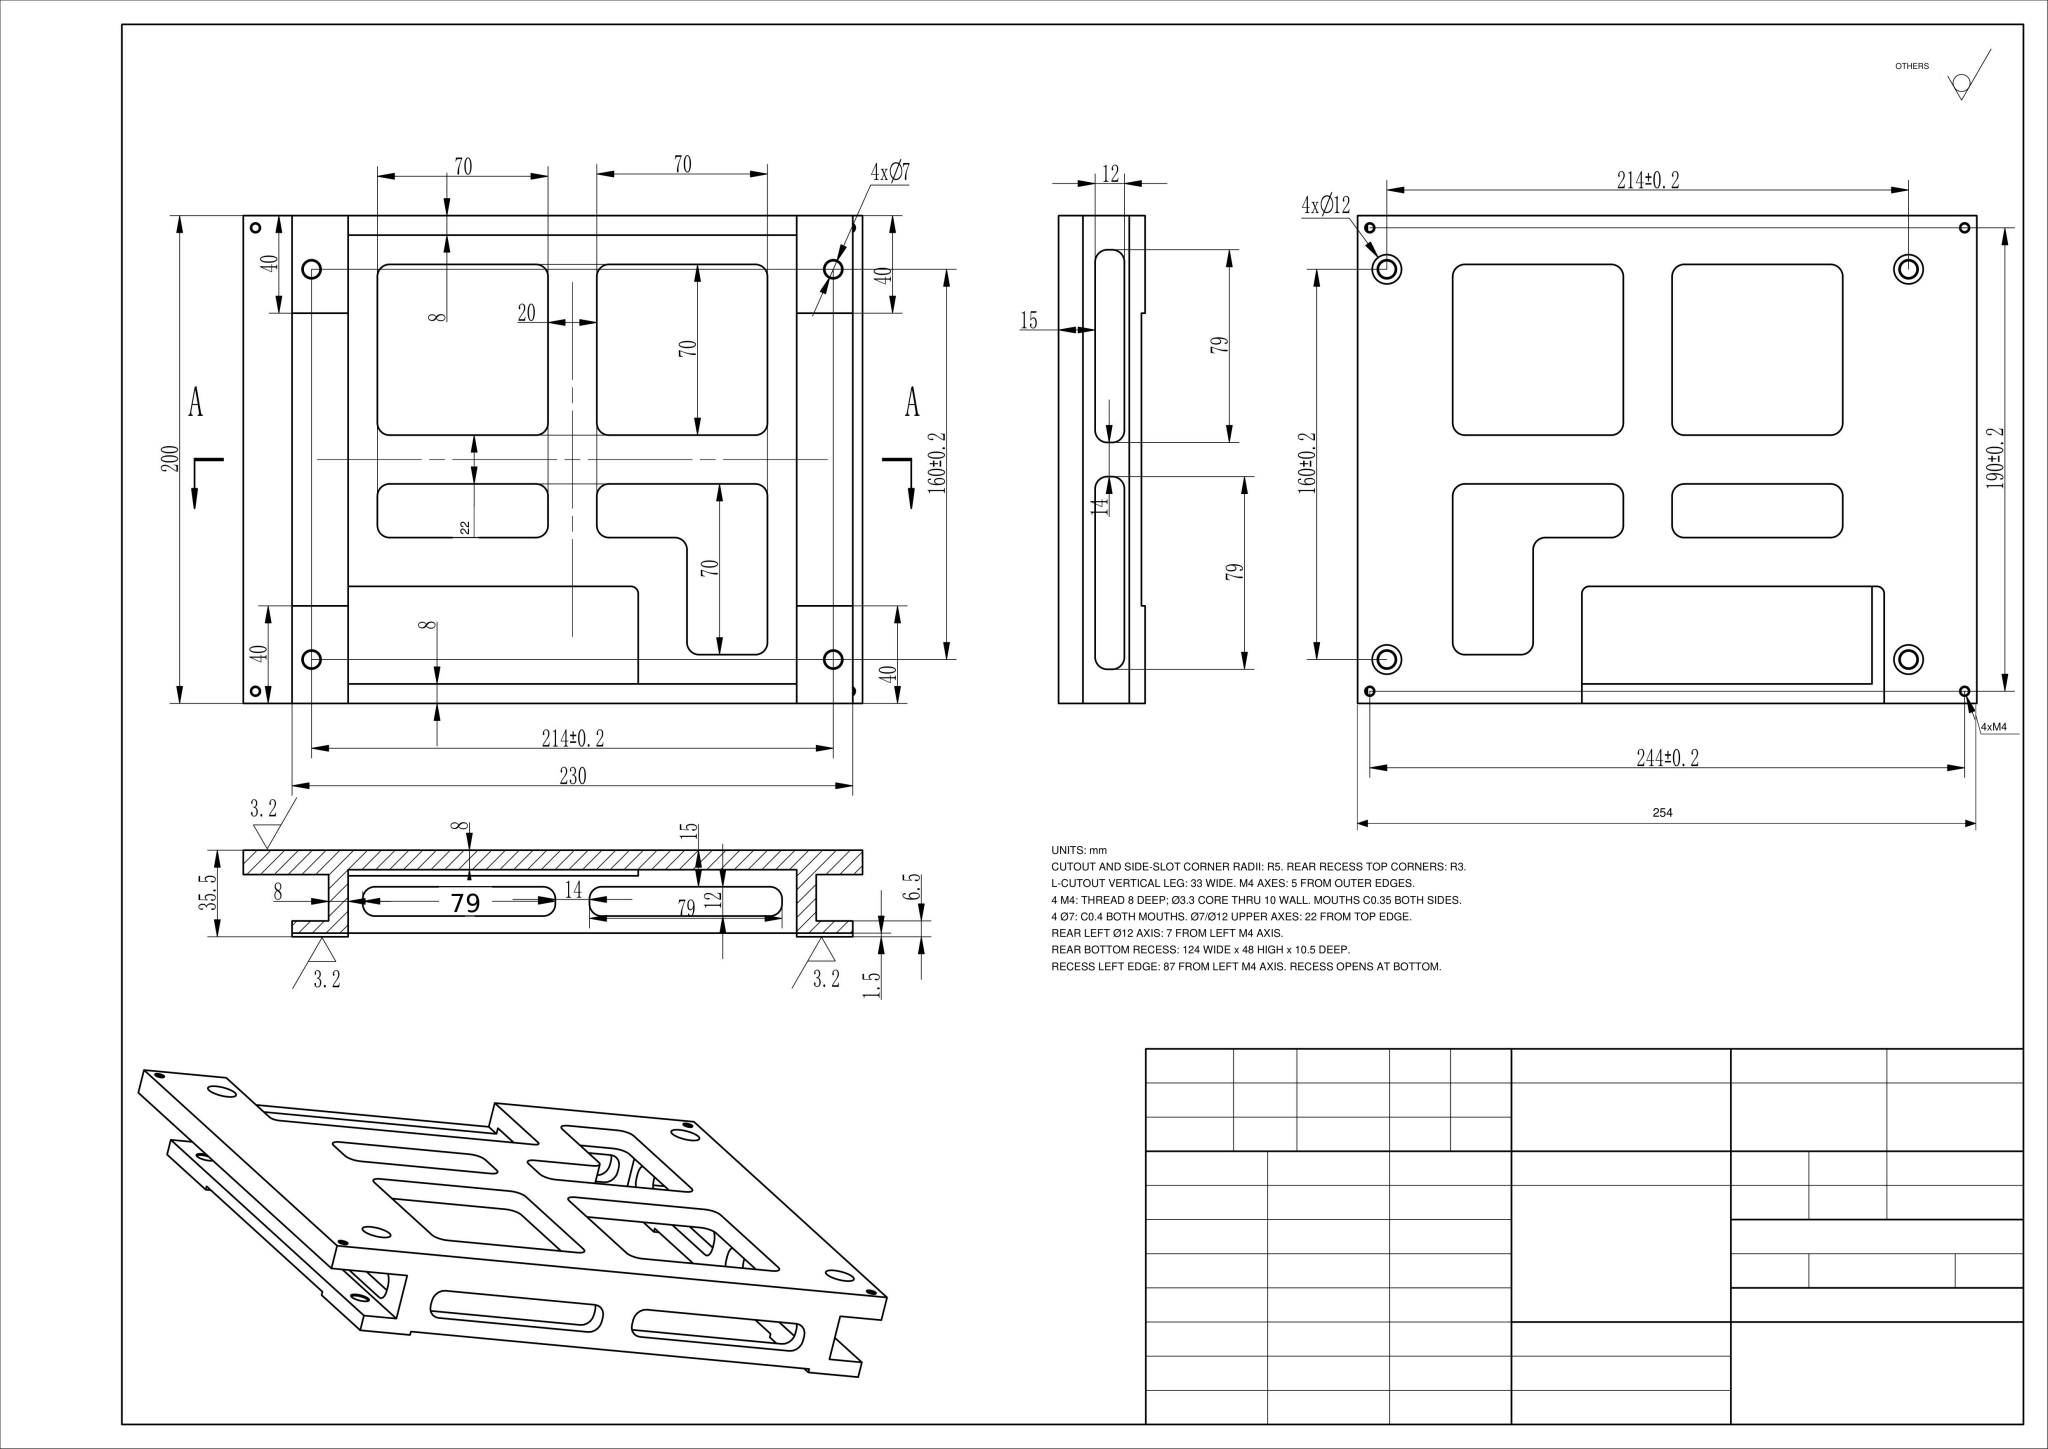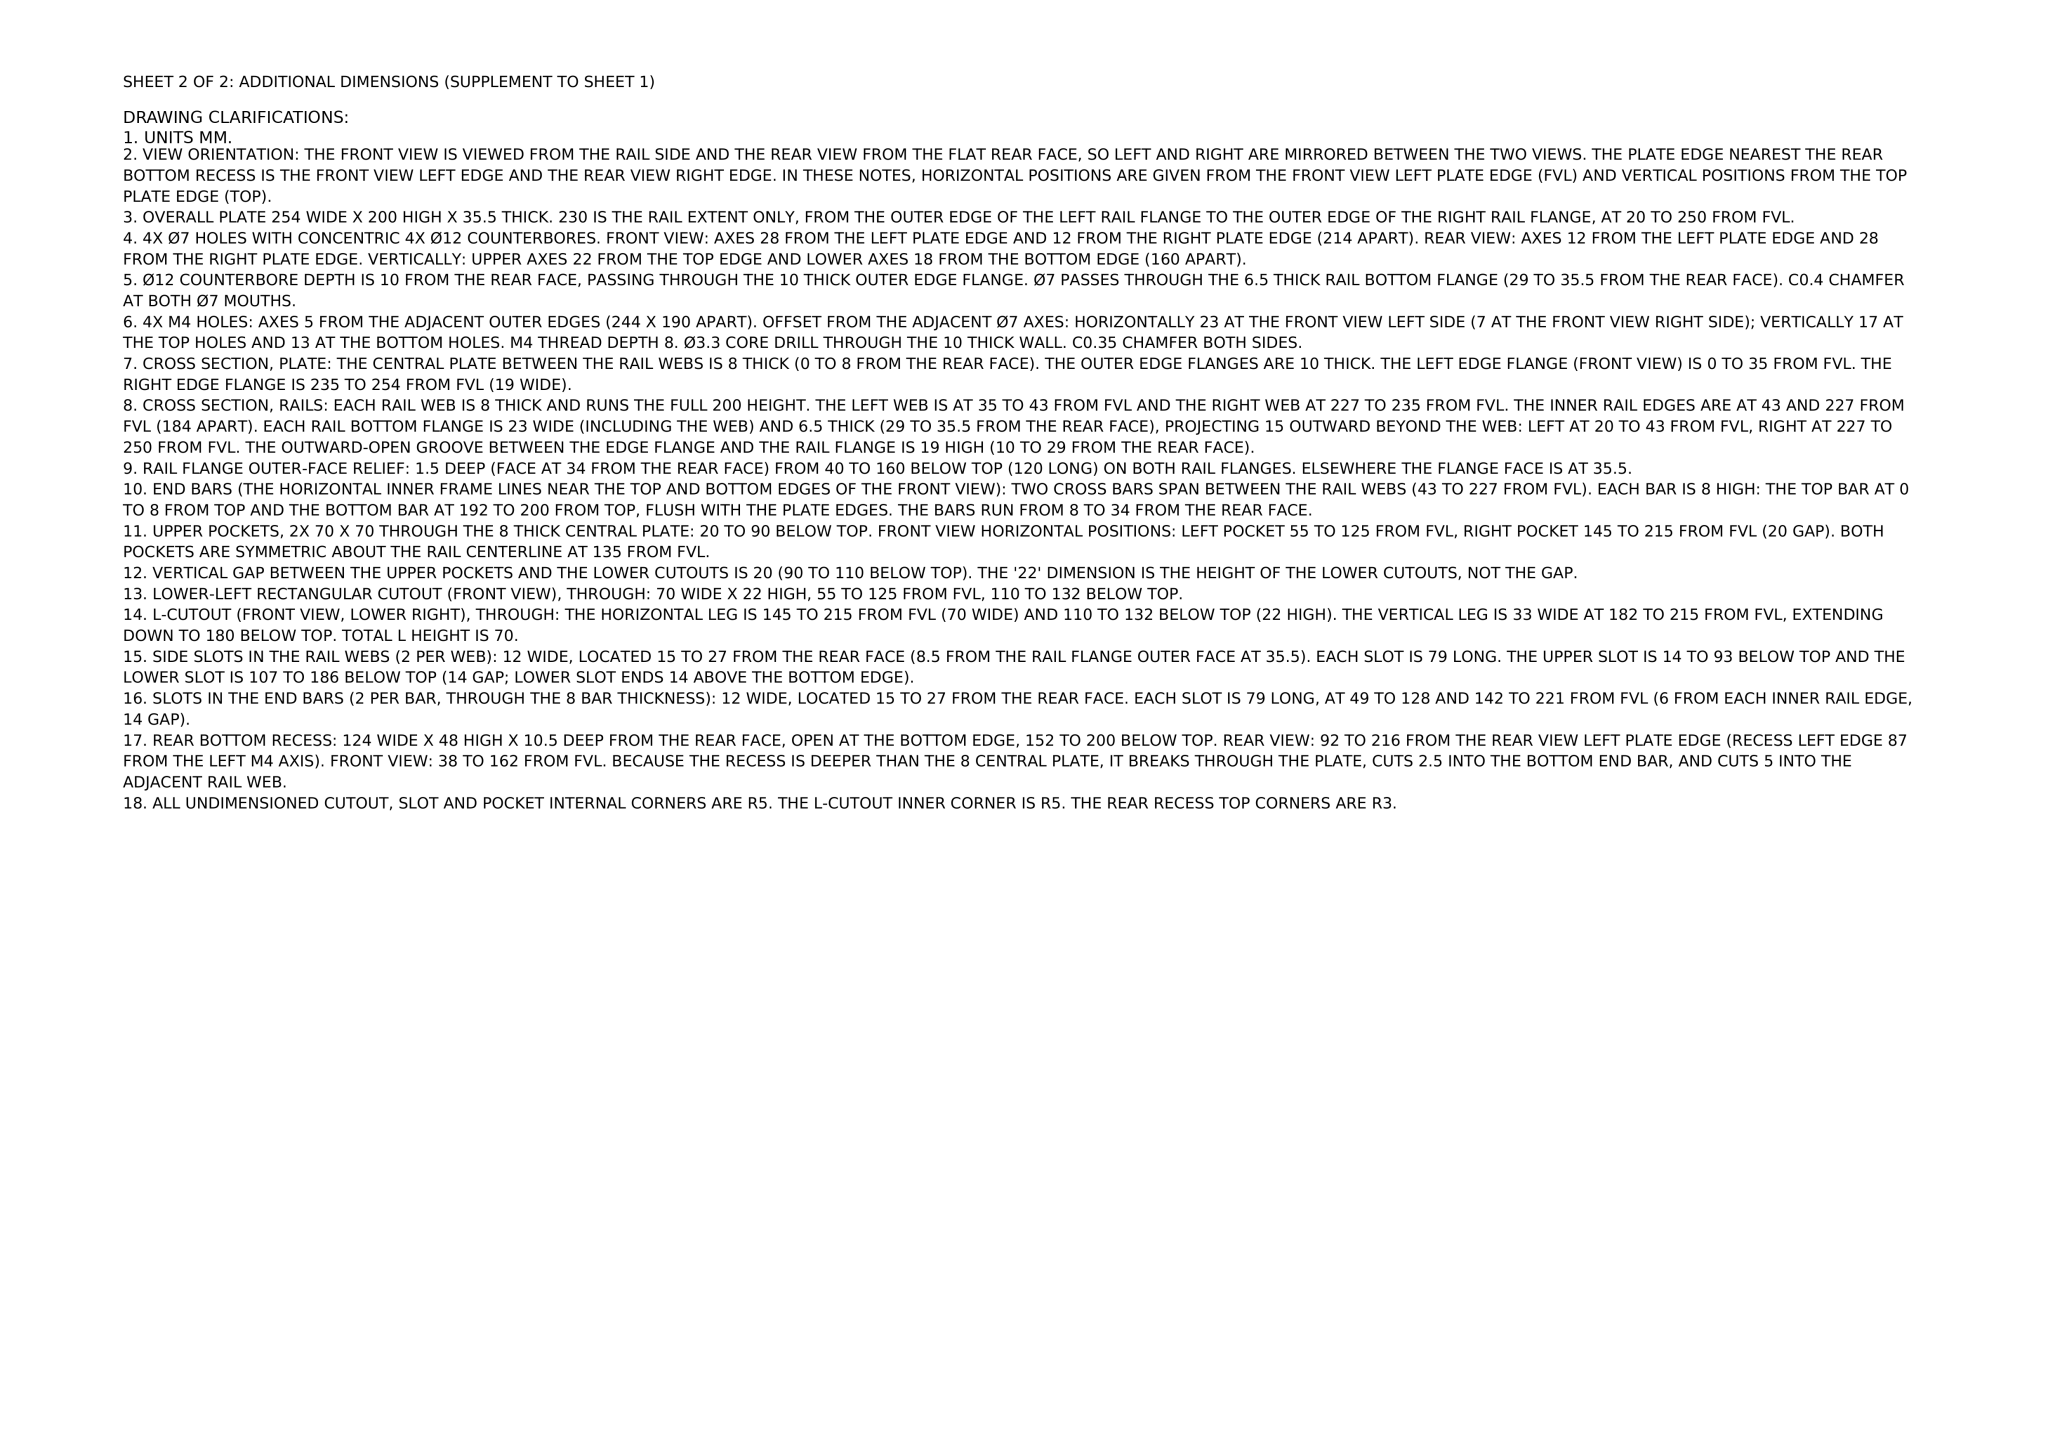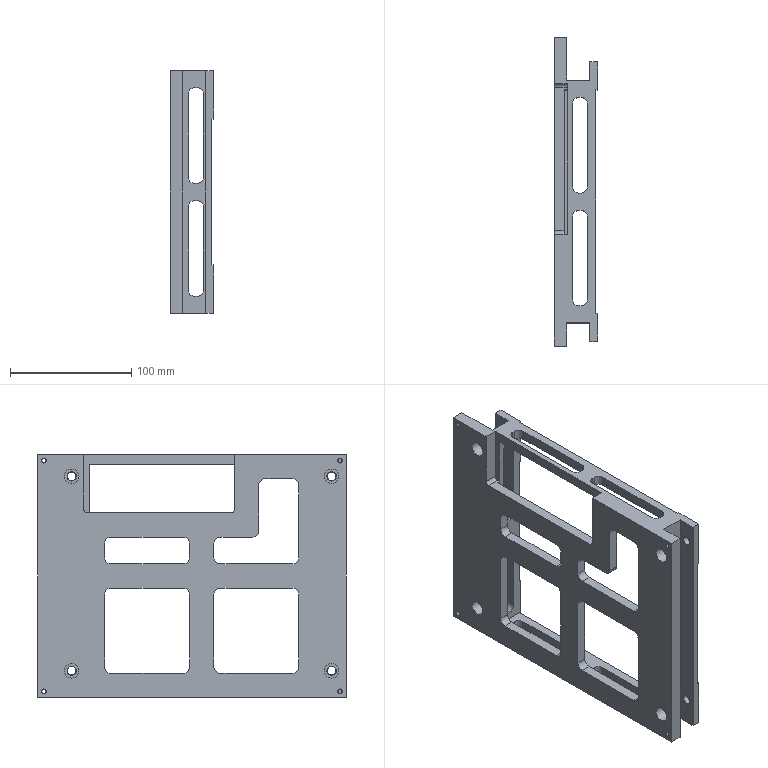Part | NX | mm | 1 solid | 164 faces | box 35.5 x 254 x 200 mm | volume 392493 mm3 | plane 84 | cylinder 64 | cone 16 | commonest cylinder face diameters 10 x50 7 x4 12 x4 3.3 x4 6 x2